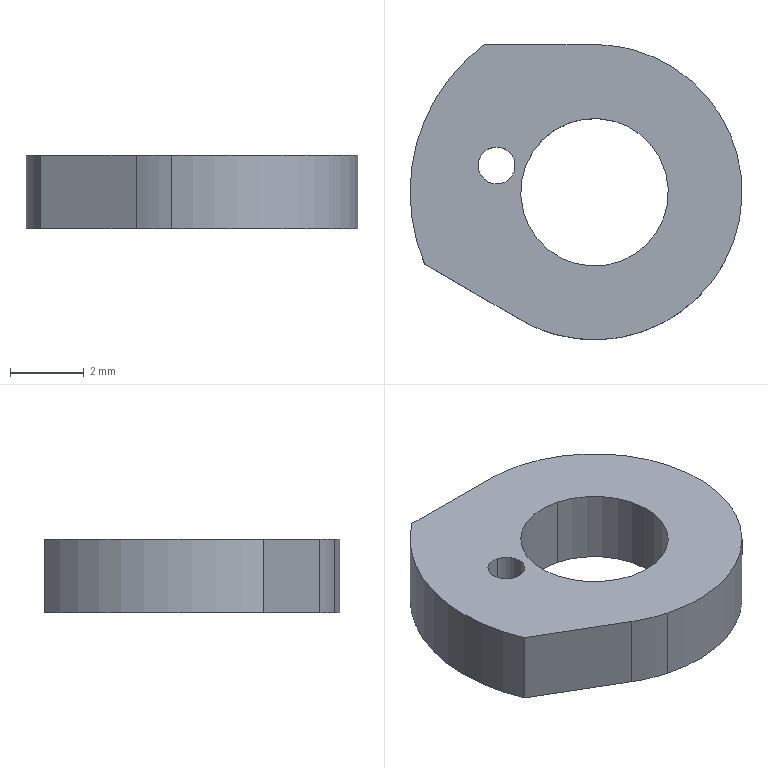Component | SolidWorks | EccentricCam(Front)-4 | 1 solid | 12 faces | box 9 x 8.01 x 2 mm | volume 89 mm3 | cylinder 8 | plane 4 | commonest cylinder face diameters 8 x3 1 x2 4 x2 10 x1
build123d program:
from build123d import *

# Parameters (mm, degrees)
SKETCH1_R           = 2
SKETCH1_R_2         = 0.5
BOSS_EXTRUDE1_DEPTH = 2


with BuildPart() as part:
    # Sketch1 → Boss-Extrude1 (new body)
    with BuildSketch(Plane.XY):
        with BuildLine():
            Line((-13.864, -1.465), (-13.087, 1.433))
            ThreePointArc((-13.087, 1.433), (-10, 2.5), (-6.913, 1.433))
            Line((-6.913, 1.433), (-6.136, -1.465))
            ThreePointArc((-6.136, -1.465), (-10, -6.5), (-13.864, -1.465))
        make_face()
        with Locations((-10, -2.5)):
            Circle(SKETCH1_R, mode=Mode.SUBTRACT)
        with Locations((-10, 0.25)):
            Circle(SKETCH1_R_2, mode=Mode.SUBTRACT)
    extrude(amount=BOSS_EXTRUDE1_DEPTH)


solid = part.part

# Placed as in the assembly
solid = solid.moved(Location((-9.78, 7.805, -5), (0, 0, 74.742)))
STEP:
#1=CARTESIAN_POINT('',(-0.4351,-0.2504,-0.1969));
#2=VERTEX_POINT('',#1);
#3=CARTESIAN_POINT('',(-0.4731,-0.2345,-0.1969));
#4=VERTEX_POINT('',#3);
#5=CARTESIAN_POINT('',(-0.3937,-0.09843,-0.1969));
#6=DIRECTION('',(0.,0.,-1.));
#7=DIRECTION('',(-0.2632,-0.9648,-0.));
#8=AXIS2_PLACEMENT_3D('',#5,#6,#7);
#9=CIRCLE('',#8,0.1575);
#10=EDGE_CURVE('',#2,#4,#9,.T.);
#11=ORIENTED_EDGE('',*,*,#10,.F.);
#12=CARTESIAN_POINT('',(-0.4351,-0.2504,-0.1181));
#13=VERTEX_POINT('',#12);
#14=CARTESIAN_POINT('',(-0.4351,-0.2504,-0.1969));
#15=DIRECTION('',(-0.,-0.,1.));
#16=VECTOR('',#15,39.37);
#17=LINE('',#14,#16);
#18=EDGE_CURVE('',#2,#13,#17,.T.);
#19=ORIENTED_EDGE('',*,*,#18,.T.);
#20=CARTESIAN_POINT('',(-0.4731,-0.2345,-0.1181));
#21=VERTEX_POINT('',#20);
#22=CARTESIAN_POINT('',(-0.3937,-0.09843,-0.1181));
#23=DIRECTION('',(0.,0.,-1.));
#24=DIRECTION('',(-0.2632,-0.9648,-0.));
#25=AXIS2_PLACEMENT_3D('',#22,#23,#24);
#26=CIRCLE('',#25,0.1575);
#27=EDGE_CURVE('',#13,#21,#26,.T.);
#28=ORIENTED_EDGE('',*,*,#27,.T.);
#29=CARTESIAN_POINT('',(-0.4731,-0.2345,-0.1969));
#30=DIRECTION('',(-0.,-0.,1.));
#31=VECTOR('',#30,39.37);
#32=LINE('',#29,#31);
#33=EDGE_CURVE('',#4,#21,#32,.T.);
#34=ORIENTED_EDGE('',*,*,#33,.F.);
#35=EDGE_LOOP('',(#11,#19,#28,#34));
#36=FACE_OUTER_BOUND('',#35,.T.);
#37=CARTESIAN_POINT('',(-0.3937,-0.09843,-0.1969));
#38=DIRECTION('',(-0.,-0.,1.));
#39=DIRECTION('',(0.2632,0.9648,0.));
#40=AXIS2_PLACEMENT_3D('',#37,#38,#39);
#41=CYLINDRICAL_SURFACE('',#40,0.1575);
#42=ADVANCED_FACE('',(#36),#41,.T.);
#43=ORIENTED_EDGE('',*,*,#18,.F.);
#44=CARTESIAN_POINT('',(-0.3523,0.0535,-0.1969));
#45=VERTEX_POINT('',#44);
#46=CARTESIAN_POINT('',(-0.3937,-0.09843,-0.1969));
#47=DIRECTION('',(0.,0.,-1.));
#48=DIRECTION('',(-0.2632,-0.9648,-0.));
#49=AXIS2_PLACEMENT_3D('',#46,#47,#48);
#50=CIRCLE('',#49,0.1575);
#51=EDGE_CURVE('',#45,#2,#50,.T.);
#52=ORIENTED_EDGE('',*,*,#51,.F.);
#53=CARTESIAN_POINT('',(-0.3523,0.0535,-0.1181));
#54=VERTEX_POINT('',#53);
#55=CARTESIAN_POINT('',(-0.3523,0.0535,-0.1969));
#56=DIRECTION('',(-0.,-0.,1.));
#57=VECTOR('',#56,39.37);
#58=LINE('',#55,#57);
#59=EDGE_CURVE('',#45,#54,#58,.T.);
#60=ORIENTED_EDGE('',*,*,#59,.T.);
#61=CARTESIAN_POINT('',(-0.3937,-0.09843,-0.1181));
#62=DIRECTION('',(0.,0.,-1.));
#63=DIRECTION('',(-0.2632,-0.9648,-0.));
#64=AXIS2_PLACEMENT_3D('',#61,#62,#63);
#65=CIRCLE('',#64,0.1575);
#66=EDGE_CURVE('',#54,#13,#65,.T.);
#67=ORIENTED_EDGE('',*,*,#66,.T.);
#68=EDGE_LOOP('',(#43,#52,#60,#67));
#69=FACE_OUTER_BOUND('',#68,.T.);
#70=CARTESIAN_POINT('',(-0.3937,-0.09843,-0.1969));
#71=DIRECTION('',(-0.,-0.,1.));
#72=DIRECTION('',(0.2632,0.9648,0.));
#73=AXIS2_PLACEMENT_3D('',#70,#71,#72);
#74=CYLINDRICAL_SURFACE('',#73,0.1575);
#75=ADVANCED_FACE('',(#69),#74,.T.);
#76=CARTESIAN_POINT('',(-0.493,-0.05094,-0.1969));
#77=VERTEX_POINT('',#76);
#78=CARTESIAN_POINT('',(-0.5033,-0.08892,-0.1969));
#79=VERTEX_POINT('',#78);
#80=CARTESIAN_POINT('',(-0.4982,-0.06993,-0.1969));
#81=DIRECTION('',(0.,0.,-1.));
#82=DIRECTION('',(-0.2632,-0.9648,-0.));
#83=AXIS2_PLACEMENT_3D('',#80,#81,#82);
#84=CIRCLE('',#83,0.01969);
#85=EDGE_CURVE('',#77,#79,#84,.T.);
#86=ORIENTED_EDGE('',*,*,#85,.T.);
#87=CARTESIAN_POINT('',(-0.5033,-0.08892,-0.1181));
#88=VERTEX_POINT('',#87);
#89=CARTESIAN_POINT('',(-0.5033,-0.08892,-0.1969));
#90=DIRECTION('',(-0.,-0.,1.));
#91=VECTOR('',#90,39.37);
#92=LINE('',#89,#91);
#93=EDGE_CURVE('',#79,#88,#92,.T.);
#94=ORIENTED_EDGE('',*,*,#93,.T.);
#95=CARTESIAN_POINT('',(-0.493,-0.05094,-0.1181));
#96=VERTEX_POINT('',#95);
#97=CARTESIAN_POINT('',(-0.4982,-0.06993,-0.1181));
#98=DIRECTION('',(0.,0.,-1.));
#99=DIRECTION('',(-0.2632,-0.9648,-0.));
#100=AXIS2_PLACEMENT_3D('',#97,#98,#99);
#101=CIRCLE('',#100,0.01969);
#102=EDGE_CURVE('',#96,#88,#101,.T.);
#103=ORIENTED_EDGE('',*,*,#102,.F.);
#104=CARTESIAN_POINT('',(-0.493,-0.05094,-0.1969));
#105=DIRECTION('',(-0.,-0.,1.));
#106=VECTOR('',#105,39.37);
#107=LINE('',#104,#106);
#108=EDGE_CURVE('',#77,#96,#107,.T.);
#109=ORIENTED_EDGE('',*,*,#108,.F.);
#110=EDGE_LOOP('',(#86,#94,#103,#109));
#111=FACE_OUTER_BOUND('',#110,.T.);
#112=CARTESIAN_POINT('',(-0.4982,-0.06993,-0.1969));
#113=DIRECTION('',(-0.,-0.,1.));
#114=DIRECTION('',(0.2632,0.9648,0.));
#115=AXIS2_PLACEMENT_3D('',#112,#113,#114);
#116=CYLINDRICAL_SURFACE('',#115,0.01969);
#117=ADVANCED_FACE('',(#111),#116,.F.);
#118=CARTESIAN_POINT('',(-0.373,-0.02246,-0.1969));
#119=VERTEX_POINT('',#118);
#120=CARTESIAN_POINT('',(-0.4144,-0.1744,-0.1969));
#121=VERTEX_POINT('',#120);
#122=CARTESIAN_POINT('',(-0.3937,-0.09843,-0.1969));
#123=DIRECTION('',(0.,0.,-1.));
#124=DIRECTION('',(-0.2632,-0.9648,-0.));
#125=AXIS2_PLACEMENT_3D('',#122,#123,#124);
#126=CIRCLE('',#125,0.07874);
#127=EDGE_CURVE('',#119,#121,#126,.T.);
#128=ORIENTED_EDGE('',*,*,#127,.T.);
#129=CARTESIAN_POINT('',(-0.4144,-0.1744,-0.1181));
#130=VERTEX_POINT('',#129);
#131=CARTESIAN_POINT('',(-0.4144,-0.1744,-0.1969));
#132=DIRECTION('',(-0.,-0.,1.));
#133=VECTOR('',#132,39.37);
#134=LINE('',#131,#133);
#135=EDGE_CURVE('',#121,#130,#134,.T.);
#136=ORIENTED_EDGE('',*,*,#135,.T.);
#137=CARTESIAN_POINT('',(-0.373,-0.02246,-0.1181));
#138=VERTEX_POINT('',#137);
#139=CARTESIAN_POINT('',(-0.3937,-0.09843,-0.1181));
#140=DIRECTION('',(0.,0.,-1.));
#141=DIRECTION('',(-0.2632,-0.9648,-0.));
#142=AXIS2_PLACEMENT_3D('',#139,#140,#141);
#143=CIRCLE('',#142,0.07874);
#144=EDGE_CURVE('',#138,#130,#143,.T.);
#145=ORIENTED_EDGE('',*,*,#144,.F.);
#146=CARTESIAN_POINT('',(-0.373,-0.02246,-0.1969));
#147=DIRECTION('',(-0.,-0.,1.));
#148=VECTOR('',#147,39.37);
#149=LINE('',#146,#148);
#150=EDGE_CURVE('',#119,#138,#149,.T.);
#151=ORIENTED_EDGE('',*,*,#150,.F.);
#152=EDGE_LOOP('',(#128,#136,#145,#151));
#153=FACE_OUTER_BOUND('',#152,.T.);
#154=CARTESIAN_POINT('',(-0.3937,-0.09843,-0.1969));
#155=DIRECTION('',(-0.,-0.,1.));
#156=DIRECTION('',(0.2632,0.9648,0.));
#157=AXIS2_PLACEMENT_3D('',#154,#155,#156);
#158=CYLINDRICAL_SURFACE('',#157,0.07874);
#159=ADVANCED_FACE('',(#153),#158,.F.);
#160=CARTESIAN_POINT('',(-0.5751,-0.1749,-0.1181));
#161=VERTEX_POINT('',#160);
#162=CARTESIAN_POINT('',(-0.4672,-0.2379,-0.1181));
#163=DIRECTION('',(-0.8638,0.5039,0.));
#164=VECTOR('',#163,39.37);
#165=LINE('',#162,#164);
#166=EDGE_CURVE('',#21,#161,#165,.T.);
#167=ORIENTED_EDGE('',*,*,#166,.T.);
#168=CARTESIAN_POINT('',(-0.5751,-0.1749,-0.1969));
#169=VERTEX_POINT('',#168);
#170=CARTESIAN_POINT('',(-0.5751,-0.1749,-0.1969));
#171=DIRECTION('',(-0.,-0.,1.));
#172=VECTOR('',#171,39.37);
#173=LINE('',#170,#172);
#174=EDGE_CURVE('',#169,#161,#173,.T.);
#175=ORIENTED_EDGE('',*,*,#174,.F.);
#176=CARTESIAN_POINT('',(-0.4672,-0.2379,-0.1969));
#177=DIRECTION('',(-0.8638,0.5039,0.));
#178=VECTOR('',#177,39.37);
#179=LINE('',#176,#178);
#180=EDGE_CURVE('',#4,#169,#179,.T.);
#181=ORIENTED_EDGE('',*,*,#180,.F.);
#182=ORIENTED_EDGE('',*,*,#33,.T.);
#183=EDGE_LOOP('',(#167,#175,#181,#182));
#184=FACE_OUTER_BOUND('',#183,.T.);
#185=CARTESIAN_POINT('',(-0.4672,-0.2379,-0.1969));
#186=DIRECTION('',(0.5039,0.8638,0.));
#187=DIRECTION('',(0.8638,-0.5039,-0.));
#188=AXIS2_PLACEMENT_3D('',#185,#186,#187);
#189=PLANE('',#188);
#190=ADVANCED_FACE('',(#184),#189,.F.);
#191=CARTESIAN_POINT('',(-0.5111,0.05958,-0.1181));
#192=VERTEX_POINT('',#191);
#193=CARTESIAN_POINT('',(-0.3937,-0.09843,-0.1181));
#194=DIRECTION('',(0.,0.,-1.));
#195=DIRECTION('',(-0.2632,-0.9648,-0.));
#196=AXIS2_PLACEMENT_3D('',#193,#194,#195);
#197=CIRCLE('',#196,0.1969);
#198=EDGE_CURVE('',#161,#192,#197,.T.);
#199=ORIENTED_EDGE('',*,*,#198,.T.);
#200=CARTESIAN_POINT('',(-0.5111,0.05958,-0.1969));
#201=VERTEX_POINT('',#200);
#202=CARTESIAN_POINT('',(-0.5111,0.05958,-0.1969));
#203=DIRECTION('',(-0.,-0.,1.));
#204=VECTOR('',#203,39.37);
#205=LINE('',#202,#204);
#206=EDGE_CURVE('',#201,#192,#205,.T.);
#207=ORIENTED_EDGE('',*,*,#206,.F.);
#208=CARTESIAN_POINT('',(-0.3937,-0.09843,-0.1969));
#209=DIRECTION('',(0.,0.,-1.));
#210=DIRECTION('',(-0.2632,-0.9648,-0.));
#211=AXIS2_PLACEMENT_3D('',#208,#209,#210);
#212=CIRCLE('',#211,0.1969);
#213=EDGE_CURVE('',#169,#201,#212,.T.);
#214=ORIENTED_EDGE('',*,*,#213,.F.);
#215=ORIENTED_EDGE('',*,*,#174,.T.);
#216=EDGE_LOOP('',(#199,#207,#214,#215));
#217=FACE_OUTER_BOUND('',#216,.T.);
#218=CARTESIAN_POINT('',(-0.3937,-0.09843,-0.1969));
#219=DIRECTION('',(-0.,-0.,1.));
#220=DIRECTION('',(0.2632,0.9648,0.));
#221=AXIS2_PLACEMENT_3D('',#218,#219,#220);
#222=CYLINDRICAL_SURFACE('',#221,0.1969);
#223=ADVANCED_FACE('',(#217),#222,.T.);
#224=CARTESIAN_POINT('',(-0.393,0.05905,-0.1181));
#225=VERTEX_POINT('',#224);
#226=CARTESIAN_POINT('',(-0.59,0.05994,-0.1181));
#227=DIRECTION('',(-1.,0.004495,0.));
#228=VECTOR('',#227,39.37);
#229=LINE('',#226,#228);
#230=EDGE_CURVE('',#225,#192,#229,.T.);
#231=ORIENTED_EDGE('',*,*,#230,.F.);
#232=CARTESIAN_POINT('',(-0.393,0.05905,-0.1969));
#233=VERTEX_POINT('',#232);
#234=CARTESIAN_POINT('',(-0.393,0.05905,-0.1969));
#235=DIRECTION('',(-0.,-0.,1.));
#236=VECTOR('',#235,39.37);
#237=LINE('',#234,#236);
#238=EDGE_CURVE('',#233,#225,#237,.T.);
#239=ORIENTED_EDGE('',*,*,#238,.F.);
#240=CARTESIAN_POINT('',(-0.59,0.05994,-0.1969));
#241=DIRECTION('',(-1.,0.004495,0.));
#242=VECTOR('',#241,39.37);
#243=LINE('',#240,#242);
#244=EDGE_CURVE('',#233,#201,#243,.T.);
#245=ORIENTED_EDGE('',*,*,#244,.T.);
#246=ORIENTED_EDGE('',*,*,#206,.T.);
#247=EDGE_LOOP('',(#231,#239,#245,#246));
#248=FACE_OUTER_BOUND('',#247,.T.);
#249=CARTESIAN_POINT('',(-0.59,0.05994,-0.1969));
#250=DIRECTION('',(0.004495,1.,0.));
#251=DIRECTION('',(1.,-0.004495,-0.));
#252=AXIS2_PLACEMENT_3D('',#249,#250,#251);
#253=PLANE('',#252);
#254=ADVANCED_FACE('',(#248),#253,.T.);
#255=ORIENTED_EDGE('',*,*,#135,.F.);
#256=CARTESIAN_POINT('',(-0.3937,-0.09843,-0.1969));
#257=DIRECTION('',(0.,0.,-1.));
#258=DIRECTION('',(-0.2632,-0.9648,-0.));
#259=AXIS2_PLACEMENT_3D('',#256,#257,#258);
#260=CIRCLE('',#259,0.07874);
#261=EDGE_CURVE('',#121,#119,#260,.T.);
#262=ORIENTED_EDGE('',*,*,#261,.T.);
#263=ORIENTED_EDGE('',*,*,#150,.T.);
#264=CARTESIAN_POINT('',(-0.3937,-0.09843,-0.1181));
#265=DIRECTION('',(0.,0.,-1.));
#266=DIRECTION('',(-0.2632,-0.9648,-0.));
#267=AXIS2_PLACEMENT_3D('',#264,#265,#266);
#268=CIRCLE('',#267,0.07874);
#269=EDGE_CURVE('',#130,#138,#268,.T.);
#270=ORIENTED_EDGE('',*,*,#269,.F.);
#271=EDGE_LOOP('',(#255,#262,#263,#270));
#272=FACE_OUTER_BOUND('',#271,.T.);
#273=CARTESIAN_POINT('',(-0.3937,-0.09843,-0.1969));
#274=DIRECTION('',(-0.,-0.,1.));
#275=DIRECTION('',(0.2632,0.9648,0.));
#276=AXIS2_PLACEMENT_3D('',#273,#274,#275);
#277=CYLINDRICAL_SURFACE('',#276,0.07874);
#278=ADVANCED_FACE('',(#272),#277,.F.);
#279=ORIENTED_EDGE('',*,*,#93,.F.);
#280=CARTESIAN_POINT('',(-0.4982,-0.06993,-0.1969));
#281=DIRECTION('',(0.,0.,-1.));
#282=DIRECTION('',(-0.2632,-0.9648,-0.));
#283=AXIS2_PLACEMENT_3D('',#280,#281,#282);
#284=CIRCLE('',#283,0.01969);
#285=EDGE_CURVE('',#79,#77,#284,.T.);
#286=ORIENTED_EDGE('',*,*,#285,.T.);
#287=ORIENTED_EDGE('',*,*,#108,.T.);
#288=CARTESIAN_POINT('',(-0.4982,-0.06993,-0.1181));
#289=DIRECTION('',(0.,0.,-1.));
#290=DIRECTION('',(-0.2632,-0.9648,-0.));
#291=AXIS2_PLACEMENT_3D('',#288,#289,#290);
#292=CIRCLE('',#291,0.01969);
#293=EDGE_CURVE('',#88,#96,#292,.T.);
#294=ORIENTED_EDGE('',*,*,#293,.F.);
#295=EDGE_LOOP('',(#279,#286,#287,#294));
#296=FACE_OUTER_BOUND('',#295,.T.);
#297=CARTESIAN_POINT('',(-0.4982,-0.06993,-0.1969));
#298=DIRECTION('',(-0.,-0.,1.));
#299=DIRECTION('',(0.2632,0.9648,0.));
#300=AXIS2_PLACEMENT_3D('',#297,#298,#299);
#301=CYLINDRICAL_SURFACE('',#300,0.01969);
#302=ADVANCED_FACE('',(#296),#301,.F.);
#303=ORIENTED_EDGE('',*,*,#59,.F.);
#304=CARTESIAN_POINT('',(-0.3937,-0.09843,-0.1969));
#305=DIRECTION('',(0.,0.,-1.));
#306=DIRECTION('',(-0.2632,-0.9648,-0.));
#307=AXIS2_PLACEMENT_3D('',#304,#305,#306);
#308=CIRCLE('',#307,0.1575);
#309=EDGE_CURVE('',#233,#45,#308,.T.);
#310=ORIENTED_EDGE('',*,*,#309,.F.);
#311=ORIENTED_EDGE('',*,*,#238,.T.);
#312=CARTESIAN_POINT('',(-0.3937,-0.09843,-0.1181));
#313=DIRECTION('',(0.,0.,-1.));
#314=DIRECTION('',(-0.2632,-0.9648,-0.));
#315=AXIS2_PLACEMENT_3D('',#312,#313,#314);
#316=CIRCLE('',#315,0.1575);
#317=EDGE_CURVE('',#225,#54,#316,.T.);
#318=ORIENTED_EDGE('',*,*,#317,.T.);
#319=EDGE_LOOP('',(#303,#310,#311,#318));
#320=FACE_OUTER_BOUND('',#319,.T.);
#321=CARTESIAN_POINT('',(-0.3937,-0.09843,-0.1969));
#322=DIRECTION('',(-0.,-0.,1.));
#323=DIRECTION('',(0.2632,0.9648,0.));
#324=AXIS2_PLACEMENT_3D('',#321,#322,#323);
#325=CYLINDRICAL_SURFACE('',#324,0.1575);
#326=ADVANCED_FACE('',(#320),#325,.T.);
#327=ORIENTED_EDGE('',*,*,#85,.F.);
#328=ORIENTED_EDGE('',*,*,#285,.F.);
#329=EDGE_LOOP('',(#327,#328));
#330=FACE_BOUND('',#329,.T.);
#331=ORIENTED_EDGE('',*,*,#127,.F.);
#332=ORIENTED_EDGE('',*,*,#261,.F.);
#333=EDGE_LOOP('',(#331,#332));
#334=FACE_BOUND('',#333,.T.);
#335=ORIENTED_EDGE('',*,*,#180,.T.);
#336=ORIENTED_EDGE('',*,*,#213,.T.);
#337=ORIENTED_EDGE('',*,*,#244,.F.);
#338=ORIENTED_EDGE('',*,*,#309,.T.);
#339=ORIENTED_EDGE('',*,*,#51,.T.);
#340=ORIENTED_EDGE('',*,*,#10,.T.);
#341=EDGE_LOOP('',(#335,#336,#337,#338,#339,#340));
#342=FACE_OUTER_BOUND('',#341,.T.);
#343=CARTESIAN_POINT('',(-0.5923,-0.4523,-0.1969));
#344=DIRECTION('',(0.,0.,-1.));
#345=DIRECTION('',(-0.2632,-0.9648,-0.));
#346=AXIS2_PLACEMENT_3D('',#343,#344,#345);
#347=PLANE('',#346);
#348=ADVANCED_FACE('',(#330,#334,#342),#347,.T.);
#349=ORIENTED_EDGE('',*,*,#102,.T.);
#350=ORIENTED_EDGE('',*,*,#293,.T.);
#351=EDGE_LOOP('',(#349,#350));
#352=FACE_BOUND('',#351,.T.);
#353=ORIENTED_EDGE('',*,*,#144,.T.);
#354=ORIENTED_EDGE('',*,*,#269,.T.);
#355=EDGE_LOOP('',(#353,#354));
#356=FACE_BOUND('',#355,.T.);
#357=ORIENTED_EDGE('',*,*,#166,.F.);
#358=ORIENTED_EDGE('',*,*,#27,.F.);
#359=ORIENTED_EDGE('',*,*,#66,.F.);
#360=ORIENTED_EDGE('',*,*,#317,.F.);
#361=ORIENTED_EDGE('',*,*,#230,.T.);
#362=ORIENTED_EDGE('',*,*,#198,.F.);
#363=EDGE_LOOP('',(#357,#358,#359,#360,#361,#362));
#364=FACE_OUTER_BOUND('',#363,.T.);
#365=CARTESIAN_POINT('',(-0.5923,-0.4523,-0.1181));
#366=DIRECTION('',(0.,0.,-1.));
#367=DIRECTION('',(-0.2632,-0.9648,-0.));
#368=AXIS2_PLACEMENT_3D('',#365,#366,#367);
#369=PLANE('',#368);
#370=ADVANCED_FACE('',(#352,#356,#364),#369,.F.);
#371=CLOSED_SHELL('',(#42,#75,#117,#159,#190,#223,#254,#278,#302,#326,#348,#370));
#372=MANIFOLD_SOLID_BREP('',#371);
#373=CARTESIAN_POINT('',(0.,0.,0.));
#374=DIRECTION('',(0.,0.,1.));
#375=DIRECTION('',(1.,0.,0.));
#376=AXIS2_PLACEMENT_3D('',#373,#374,#375);
#377=(LENGTH_UNIT()NAMED_UNIT(*)SI_UNIT($,.METRE.));
#378=LENGTH_MEASURE_WITH_UNIT(LENGTH_MEASURE(0.0254),#377);
#379=DIMENSIONAL_EXPONENTS(1.,0.,0.,0.,0.,0.,0.);
#380=(CONVERSION_BASED_UNIT('',#378)LENGTH_UNIT()NAMED_UNIT(#379));
#381=UNCERTAINTY_MEASURE_WITH_UNIT(LENGTH_MEASURE(0.00001),#380,'','');
#382=(NAMED_UNIT(*)PLANE_ANGLE_UNIT()SI_UNIT($,.RADIAN.));
#383=(NAMED_UNIT(*)SI_UNIT($,.STERADIAN.)SOLID_ANGLE_UNIT());
#384=(GEOMETRIC_REPRESENTATION_CONTEXT(3)GLOBAL_UNCERTAINTY_ASSIGNED_CONTEXT((#381))GLOBAL_UNIT_ASSIGNED_CONTEXT((#380,#382,#383))REPRESENTATION_CONTEXT('',''));
#385=ADVANCED_BREP_SHAPE_REPRESENTATION('',(#372,#376),#384);
#386=COLOUR_RGB('',0.7922,0.8196,0.9333);
#387=FILL_AREA_STYLE_COLOUR('',#386);
#388=FILL_AREA_STYLE('',(#387));
#389=SURFACE_STYLE_FILL_AREA(#388);
#390=SURFACE_SIDE_STYLE('',(#389));
#391=SURFACE_STYLE_USAGE(.BOTH.,#390);
#392=PRESENTATION_STYLE_ASSIGNMENT((#391));
#393=STYLED_ITEM('',(#392),#372);
#394=(LENGTH_UNIT()NAMED_UNIT(*)SI_UNIT($,.METRE.));
#395=LENGTH_MEASURE_WITH_UNIT(LENGTH_MEASURE(0.0254),#394);
#396=DIMENSIONAL_EXPONENTS(1.,0.,0.,0.,0.,0.,0.);
#397=(CONVERSION_BASED_UNIT('',#395)LENGTH_UNIT()NAMED_UNIT(#396));
#398=UNCERTAINTY_MEASURE_WITH_UNIT(LENGTH_MEASURE(0.00001),#397,'','');
#399=(NAMED_UNIT(*)PLANE_ANGLE_UNIT()SI_UNIT($,.RADIAN.));
#400=(NAMED_UNIT(*)SI_UNIT($,.STERADIAN.)SOLID_ANGLE_UNIT());
#401=(GEOMETRIC_REPRESENTATION_CONTEXT(3)GLOBAL_UNCERTAINTY_ASSIGNED_CONTEXT((#398))GLOBAL_UNIT_ASSIGNED_CONTEXT((#397,#399,#400))REPRESENTATION_CONTEXT('',''));
#402=MECHANICAL_DESIGN_GEOMETRIC_PRESENTATION_REPRESENTATION('',(#393),#401);
#403=PRESENTATION_LAYER_ASSIGNMENT('','',(#393));